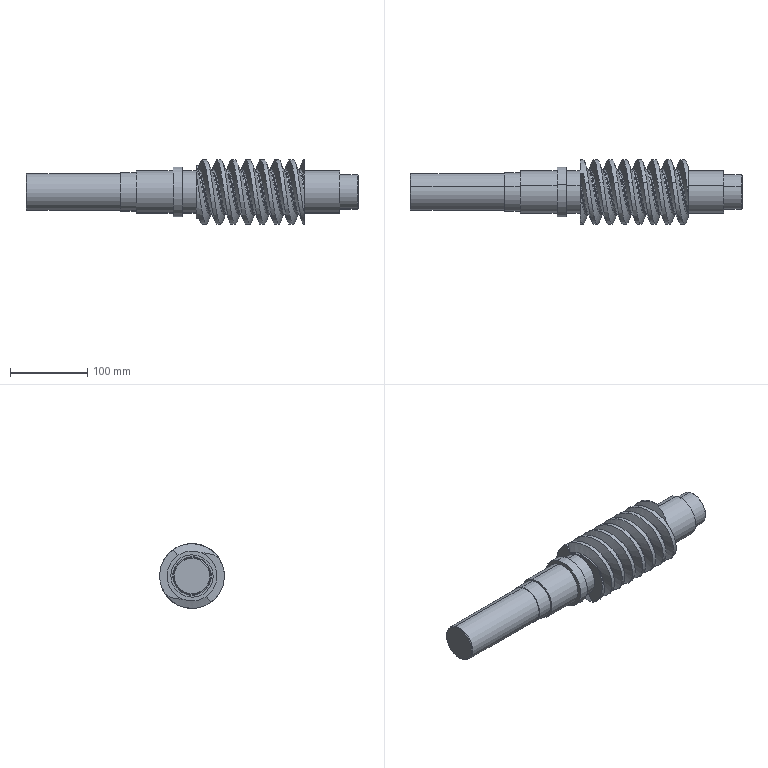Component | SolidWorks | UpperHousingAssembly-1_WormAxisAssembly-1_WormAxis-1 | 1 solid | 64 faces | volume 1175692 mm3 | cylinder 34 | plane 14 | spline 12 | cone 4 | commonest cylinder face diameters 84 x18 55 x6 45 x2 65 x2 50 x2 48 x2 14.471 x2